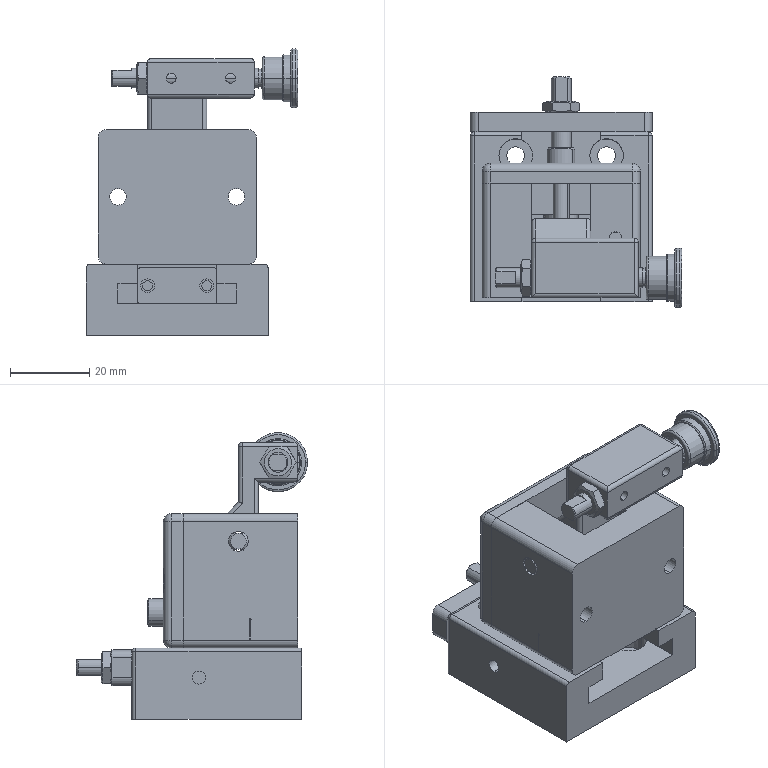Assembly | SolidWorks | mm | 14 component files | 14 solids | 1338 faces | box 53.5 x 58.5 x 72.5 mm | volume 71933 mm3 | plane 952 | cylinder 159 | spline 158 | cone 48 | sphere 13 | torus 8 | commonest cylinder face diameters 2 x27 5 x24 4 x22 4.5 x20 2.5 x12 3.3 x10 8.5 x10 4.2 x4
Bill of materials:
18M4-L16StainlessSteelScrew | 1 | SUS304 | Headed cylindrical pin or screw-like part: short cylindrical head on a plain, smooth cylindrical shank.
18M5-L35StainlessSteelScrew | 1 | SUS304 | Socket-head-screw-like part: low cylindrical head with a hexagonal recess and a long plain shank that steps down to a slightly smaller diameter near the tip.
18M5StainlessSteelNut | 2 | SUS304 | Thin hexagonal nut-like part with a plain circular through-bore and chamfered corners on both faces.
18ZTJ-NVT-01-001 | 1 | Black POM | Flanged bushing or sleeve-like part: cylindrical body, a short larger-diameter step, and a wider flange with rounded edges, all around a through-bore.
18ZTJ-NVT-01-002 | 1 | Chrome Plated Rod | Long headed pin: thin disc head on a slender cylindrical shank with a small groove near the head and a modified tip region.
18Spring1.0-15 | 1 | SKD11 | Helical coil spring-like part made of round wire, with a constant coil diameter and open ends.
18ZTJ-NVT-01-003 | 1 | #45 | Straight rod with chamfered ends and two opposing flats running its full length (double-D cross-section).
18ZTJ-NVT-01-004 | 1 | #45 | T-shaped or L-shaped block bracket: a rectangular crossbar on top of a narrower vertical leg, with several through-holes and slightly rounded edges.
18ZTJ-NVT-01-005 | 1 | #45 | Block with an open U-shaped slot, several holes on different faces, and a narrower stepped tab on one end.
18ZTJ-NVT-01-006 | 1 | #45 | Flat rectangular plate with rounded corners and edges and three plain through-holes.
18ZTJ-NVT-01-009 | 1 | #45 | Rectangular block with an inverted-T-shaped slot running through it, four vertical holes with counterbores, and one cross-hole.
18ZTJ-NVT-01-011 | 1 | #45 | Flat bar or link with rounded corners and three through-holes in a line.
1ZTJ-NVT-01-011-1 | 1 | #45 | Rectangular block that is U-shaped (C-shaped) in plan. A rectangular cutout goes through the full height in the middle of one long side, leaving a thinner central web between two full-depth end sections. Each end section has one round through hole running front to back, perpendicular to the large front face. The four outer edges that run parallel to the hole axes are rounded.
Mates:
1. coincident | 18ZTJ-NVT-01-009-1 face at (-36.6, -20.53, 84) dir (0, 0, 1) | 18ZTJ-NVT-01-005-1 face at (-33.6, -30.53, 84) dir (0, 0, -1)
2. width | 18ZTJ-NVT-01-005-1 face at (6.4, -30.53, 118) dir (1, 0, 0) | 18ZTJ-NVT-01-005-1 face at (-33.6, -30.53, 118) dir (-1, 0, 0) | 18ZTJ-NVT-01-009-1 face at (-36.6, -20.53, 84) dir (-1, 0, 0) | 18ZTJ-NVT-01-009-1 face at (9.4, -20.53, 84) dir (1, 0, 0)
3. distance | 18ZTJ-NVT-01-009-1 face at (-36.6, 22.47, 84) dir (0, 1, 0) | 18ZTJ-NVT-01-005-1 face at (-33.6, 9.47, 118) dir (0, 1, 0)
4. concentric | 18ZTJ-NVT-01-005-1 face at (-33.6, -4.53, 111) dir (-1, 0, 0) r 2.5 | 18ZTJ-NVT-01-003-1 face at (-33.6, -4.53, 111) dir (1, 0, 0) r 2.5
5. parallel | 18ZTJ-NVT-01-003-1 face at (-33.6, -6.03, 113) dir (0, 0, 1) | 18ZTJ-NVT-01-005-1 face at (-33.6, -30.53, 118) dir (0, 0, 1)
6. width | 18ZTJ-NVT-01-003-1 face at (6.4, -4.53, 111) dir (1, 0, 0) | 18ZTJ-NVT-01-003-1 face at (-33.6, -4.53, 111) dir (-1, 0, 0) | 18ZTJ-NVT-01-005-1 face at (-33.6, -30.53, 118) dir (-1, 0, 0) | 18ZTJ-NVT-01-005-1 face at (6.4, -30.53, 118) dir (1, 0, 0)
7. width | 18ZTJ-NVT-01-004-1 face at (-6.1, -19.53, 86) dir (1, 0, 0) | 18ZTJ-NVT-01-004-1 face at (-21.1, -19.53, 136) dir (-1, 0, 0) | 18ZTJ-NVT-01-005-1 face at (-21.1, 9.47, 84) dir (1, 0, 0) | 18ZTJ-NVT-01-005-1 face at (-6.1, 9.47, 84) dir (-1, 0, 0)
8. concentric | 18ZTJ-NVT-01-003-1 face at (-33.6, -4.53, 111) dir (1, 0, 0) r 2.5 | 18ZTJ-NVT-01-004-1 face at (-6.1, -4.53, 111) dir (1, 0, 0) r 2.5
9. angle | 18ZTJ-NVT-01-004-1 face at (5.9, 0.4702, 136) dir (0, 1, 0) | 18ZTJ-NVT-01-005-1 face at (-33.6, 9.47, 118) dir (0, 1, 0)
10. coincident | 18ZTJ-NVT-01-005-1 face at (-33.6, 9.47, 118) dir (0, 1, 0) | 18ZTJ-NVT-01-006-1 face at (-33.6, 9.47, 118) dir (0, -1, 0)
11. concentric | 18ZTJ-NVT-01-005-1 face at (1.4, 9.47, 101) dir (0, 1, 0) r 2.1 | 18ZTJ-NVT-01-006-1 face at (1.4, 14.47, 101) dir (0, 1, 0) r 2.25
12. concentric | 18ZTJ-NVT-01-005-1 face at (-28.6, 9.47, 101) dir (0, 1, 0) r 2.1 | 18ZTJ-NVT-01-006-1 face at (-28.6, 14.47, 101) dir (0, 1, 0) r 2.25
13. concentric | 18MTOSC80BatteryCellCornerFoldingRollerAssembly-1/18ZTJ-NVT-01-002-1 face at (14.9, -14.53, 131) dir (-1, 0, 0) r 2.5 | 18ZTJ-NVT-01-004-1 face at (5.9, -14.53, 131) dir (1, 0, 0) r 2.5
14. distance | 18MTOSC80BatteryCellCornerFoldingRollerAssembly-1/18ZTJ-NVT-01-001-1 face at (7.9, -9.03, 131) dir (-1, 0, 0) | 18ZTJ-NVT-01-004-1 face at (5.9, -19.53, 136) dir (1, 0, 0)
15. concentric | 18ZTJ-NVT-01-006-1 face at (-13.6, 14.47, 93) dir (0, 1, 0) r 2 | 18M4-L16StainlessSteelScrew-1 face at (-13.6, -1.53, 93) dir (0, 1, 0) r 2
16. coincident | 18ZTJ-NVT-01-006-1 face at (-33.6, 14.47, 118) dir (0, 1, 0) | 18M4-L16StainlessSteelScrew-1 face at (-15.514, 14.47, 95.93) dir (0, -1, 0)
17. coincident | 18ZTJ-NVT-01-009-1 face at (-36.6, 22.47, 84) dir (0, 1, 0) | 18ZTJ-NVT-01-011-1 face at (-36.6, 22.47, 83.5) dir (0, -1, 0)
18. width | 18ZTJ-NVT-01-009-1 face at (-36.6, -20.53, 84) dir (0, 0, 1) | 18ZTJ-NVT-01-009-1 face at (-28.6, -20.53, 74) dir (0, 0, 1) | 18ZTJ-NVT-01-011-1 face at (-13.6, 27.47, 79) dir (0, 1, 0) r 2.5
19. concentric | 18M5-L35StainlessSteelScrew-1 face at (-13.6, 36.47, 79) dir (0, -1, 0) r 2.5 | 18ZTJ-NVT-01-005-1 face at (-13.6, 9.47, 79) dir (0, 1, 0) r 2.5
20. coincident | 18ZTJ-NVT-01-005-1 face at (1.4, 1.47, 120.62) dir (0, -1, 0) | 18M5-L35StainlessSteelScrew-1 face at (-13.6, 1.47, 83.25) dir (0, 1, 0)
21. concentric | 18M5-L35StainlessSteelScrew-1 face at (-13.6, 36.47, 79) dir (0, -1, 0) r 2.5 | 18M5StainlessSteelNut-1 face at (-13.6, 30.17, 79) dir (0, -1, 0) r 2.5
22. coincident | 18ZTJ-NVT-01-011-1 face at (-36.6, 27.47, 83.5) dir (0, 1, 0) | 18M5StainlessSteelNut-1 face at (-13.6, 27.47, 79) dir (0, -1, 0)
23. parallel | 18ZTJ-NVT-01-011-1 face at (-36.6, 27.47, 83.5) dir (0, 0, 1) | 18M5-L35StainlessSteelScrew-1 face at (-12.1, 27.47, 81) dir (0, 0, 1)
24. parallel | 18ZTJ-NVT-01-011-1 face at (-36.6, 27.47, 83.5) dir (0, 0, 1) | 18M5StainlessSteelNut-1 face at (-11.29, 27.47, 83) dir (0, 0, 1)
25. concentric | 18ZTJ-NVT-01-009-1 face at (-32.6, 22.47, 79) dir (0, 1, 0) r 1.65 | 18ZTJ-NVT-01-011-1 face at (-32.6, 27.47, 79) dir (0, 1, 0) r 2.25
26. concentric | 18ZTJ-NVT-01-005-1 face at (-13.6, -18.53, 93) dir (0, 1, 0) r 2.9 | 18Spring1.0-15-1 sketch segment at (-13.6, -18.53, 93) dir (0, 1, 0) r 2.5
27. coincident | 18ZTJ-NVT-01-005-1 face at (-13.6, -18.53, 93) dir (0, 1, 0) | 18Spring1.0-15-1 face at (-13.6, -18.53, 93) dir (0, 1, 0)
28. concentric | 18MTOSC80BatteryCellCornerFoldingRollerAssembly-1/18ZTJ-NVT-01-002-1 face at (14.9, -14.53, 131) dir (-1, 0, 0) r 2.5 | 18M5StainlessSteelNut-2 face at (-21.1, -14.53, 131) dir (-1, 0, 0) r 2.5
29. coincident | 18ZTJ-NVT-01-004-1 face at (-21.1, -19.53, 136) dir (-1, 0, 0) | 18M5StainlessSteelNut-2 face at (-21.1, -14.53, 131) dir (1, 0, 0)
30. parallel | 18ZTJ-NVT-01-004-1 face at (5.9, -19.53, 136) dir (0, 0, 1) | 18M5StainlessSteelNut-2 face at (-23.8, -16.839, 135) dir (0, 0, 1)
31. coincident | 18ZTJ-NVT-01-005-1 face at (1.4, 1.47, 120.62) dir (0, -1, 0) | 1ZTJ-NVT-01-011-1-1 face at (-23.6, 1.47, 83) dir (0, 1, 0)
32. coincident | 18ZTJ-NVT-01-005-1 face at (-28.6, 9.47, 74) dir (0, 0, -1) | 1ZTJ-NVT-01-011-1-1 face at (-23.6, 1.47, 74) dir (0, 0, -1)
33. width | 1ZTJ-NVT-01-011-1-1 face at (-23.6, 1.47, 83) dir (-1, 0, 0) | 1ZTJ-NVT-01-011-1-1 face at (-3.6, 1.47, 83) dir (1, 0, 0) | 18ZTJ-NVT-01-005-1 face at (1.4, 9.47, 79) dir (1, 0, 0) | 18ZTJ-NVT-01-005-1 face at (-28.6, 9.47, 79) dir (-1, 0, 0)
34. coincident | 18ZTJ-NVT-01-001-1 face at (-2.611, 0.1893, 12.5) dir (0, 0, -1) | 18ZTJ-NVT-01-002-1 face at (-2.611, 0.1893, 12.5) dir (0, 0, 1)